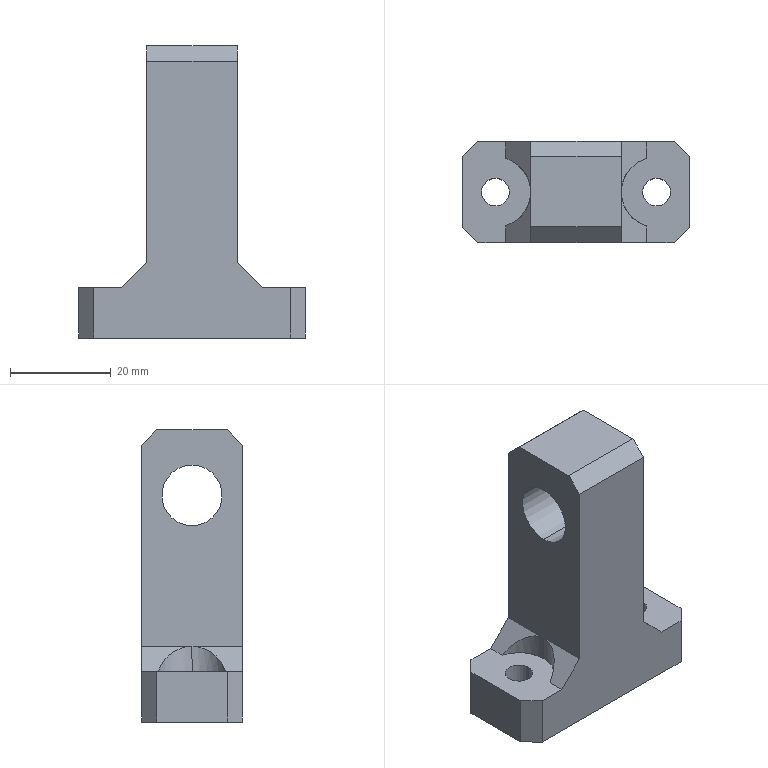Component | SolidWorks | FlipMechanismA-08-1 | 1 solid | 29 faces | box 45 x 20 x 58 mm | volume 23722 mm3 | plane 20 | cylinder 9 | commonest cylinder face diameters 5.5 x4 14 x3 12 x2
build123d program:
from build123d import *

# Parameters (mm, degrees)
SKETCH1_W                         = 10
SKETCH1_H                         = 45
EXTRUDE1_DEPTH                    = 10
SKETCH4_W                         = 18
SKETCH4_H                         = 20
EXTRUDE3_DEPTH                    = 48
M12X1_25_TAPPED_HOLE1_D           = 10.8
CHAMFER1_SIZE                     = 3
CHAMFER2_SIZE                     = 5
CHAMFER3_SIZE                     = 3
M5_CLEARANCE_HOLE_1_D             = 5.5
M5_CLEARANCE_HOLE_1_DEPTH         = 15
M5_CLEARANCE_HOLE_1_TIP           = 1.652
SKETCH4_2_R                       = 7
CUT_EXTRUDE1_DEPTH                = 18
TAPPEDHOLEMAJORDIA_M12_DEPTH      = 59.44
TAPPEDHOLEMAJORDIA_M12_DEPTH_BACK = 59.44
SKETCH7_R                         = 6


with BuildPart() as part:
    # Sketch1 → Extrude1 (new, symmetric)
    with BuildSketch(Plane(origin=(0, 0, 0), x_dir=(1, 0, 0), z_dir=(0, 1, 0))):
        Rectangle(SKETCH1_W, SKETCH1_H)
    extrude(amount=EXTRUDE1_DEPTH, both=True)

    # Sketch4 → Extrude3 (add)
    with BuildSketch(Plane(origin=(5, 0, 0), x_dir=(0, 0, -1), z_dir=(1, 0, 0))):
        Rectangle(SKETCH4_W, SKETCH4_H)
    extrude(amount=EXTRUDE3_DEPTH)

    # M12x1.25 Tapped Hole1 (through all)
    with Locations(Plane.XY.offset(9)):
        with Locations((40, 0)):
            Hole(M12X1_25_TAPPED_HOLE1_D / 2)

    # Chamfer1
    chamfer1_edges = [part.edges().sort_by_distance(p)[0] for p in [
        (0, -10, 22.5),
        (0, 10, 22.5),
        (0, -10, -22.5),
        (0, 10, -22.5),
    ]]
    chamfer(chamfer1_edges, length=CHAMFER1_SIZE)

    # Chamfer2
    chamfer2_edges = [part.edges().sort_by_distance(p)[0] for p in [
        (5, 0, -9),
        (5, 0, 9),
    ]]
    chamfer(chamfer2_edges, length=CHAMFER2_SIZE)

    # Chamfer3
    chamfer3_edges = [part.edges().sort_by_distance(p)[0] for p in [
        (53, -10, 0),
        (53, 10, 0),
    ]]
    chamfer(chamfer3_edges, length=CHAMFER3_SIZE)

    # M5 Clearance Hole 1
    with Locations(Plane(origin=(-5, 0, -16), x_dir=(0, 0, -1), z_dir=(-1, 0, 0))):
        with Locations((0, 0), (-32, 0)):
            Hole(M5_CLEARANCE_HOLE_1_D / 2, depth=M5_CLEARANCE_HOLE_1_DEPTH)
            with Locations((0, 0, -(M5_CLEARANCE_HOLE_1_DEPTH + M5_CLEARANCE_HOLE_1_TIP / 2))):  # 118° drill point
                Cone(0, M5_CLEARANCE_HOLE_1_D / 2, M5_CLEARANCE_HOLE_1_TIP, mode=Mode.SUBTRACT)

    # Sketch4_2 → Cut-Extrude1 (cut)
    with BuildSketch(Plane(origin=(5, 0, 0), x_dir=(0, 0, -1), z_dir=(1, 0, 0))):
        with Locations((16, 0)):
            Circle(SKETCH4_2_R)
        with Locations((-16, 0)):
            Circle(SKETCH4_2_R)
    extrude(amount=CUT_EXTRUDE1_DEPTH, mode=Mode.SUBTRACT)

    # Sketch7 → TappedHoleMajorDia_M12 (cut, two sides: drawn at the far end of the back side and taken through both)
    with BuildSketch(Plane.XY.offset(-TAPPEDHOLEMAJORDIA_M12_DEPTH_BACK)):
        with Locations((40, 0)):
            Circle(SKETCH7_R)
    extrude(amount=TAPPEDHOLEMAJORDIA_M12_DEPTH + TAPPEDHOLEMAJORDIA_M12_DEPTH_BACK, mode=Mode.SUBTRACT)


solid = part.part

# Placed as in the assembly
solid = solid.moved(Location((-99, 0, -40), (0, -90, 0)))
STEP:
#1=CARTESIAN_POINT('',(-4.252,-0.,-0.2362));
#2=VERTEX_POINT('',#1);
#3=CARTESIAN_POINT('',(-4.252,-0.,0.2362));
#4=VERTEX_POINT('',#3);
#5=CARTESIAN_POINT('',(-4.252,-0.,0.));
#6=DIRECTION('',(1.,0.,0.));
#7=DIRECTION('',(0.,1.,-0.));
#8=AXIS2_PLACEMENT_3D('',#5,#6,#7);
#9=CIRCLE('',#8,0.2362);
#10=EDGE_CURVE('',#2,#4,#9,.T.);
#11=ORIENTED_EDGE('',*,*,#10,.F.);
#12=CARTESIAN_POINT('',(-3.543,-0.,-0.2362));
#13=VERTEX_POINT('',#12);
#14=CARTESIAN_POINT('',(-4.783,-0.,-0.2362));
#15=DIRECTION('',(1.,-0.,0.));
#16=VECTOR('',#15,39.37);
#17=LINE('',#14,#16);
#18=EDGE_CURVE('',#2,#13,#17,.T.);
#19=ORIENTED_EDGE('',*,*,#18,.T.);
#20=CARTESIAN_POINT('',(-3.543,-0.,0.2362));
#21=VERTEX_POINT('',#20);
#22=CARTESIAN_POINT('',(-3.543,-0.,0.));
#23=DIRECTION('',(-1.,0.,-0.));
#24=DIRECTION('',(0.,-1.,0.));
#25=AXIS2_PLACEMENT_3D('',#22,#23,#24);
#26=CIRCLE('',#25,0.2362);
#27=EDGE_CURVE('',#21,#13,#26,.T.);
#28=ORIENTED_EDGE('',*,*,#27,.F.);
#29=CARTESIAN_POINT('',(-4.783,-0.,0.2362));
#30=DIRECTION('',(1.,-0.,0.));
#31=VECTOR('',#30,39.37);
#32=LINE('',#29,#31);
#33=EDGE_CURVE('',#4,#21,#32,.T.);
#34=ORIENTED_EDGE('',*,*,#33,.F.);
#35=EDGE_LOOP('',(#11,#19,#28,#34));
#36=FACE_OUTER_BOUND('',#35,.T.);
#37=CARTESIAN_POINT('',(-4.783,-0.,0.));
#38=DIRECTION('',(1.,-0.,0.));
#39=DIRECTION('',(0.,0.,1.));
#40=AXIS2_PLACEMENT_3D('',#37,#38,#39);
#41=CYLINDRICAL_SURFACE('',#40,0.2362);
#42=ADVANCED_FACE('',(#36),#41,.F.);
#43=CARTESIAN_POINT('',(-4.449,-0.2641,-1.378));
#44=VERTEX_POINT('',#43);
#45=CARTESIAN_POINT('',(-4.252,-0.,-1.181));
#46=VERTEX_POINT('',#45);
#47=CARTESIAN_POINT('',(-4.449,-0.2641,-1.378));
#48=CARTESIAN_POINT('',(-4.328,-0.228,-1.257));
#49=CARTESIAN_POINT('',(-4.252,-0.1265,-1.181));
#50=CARTESIAN_POINT('',(-4.252,-0.,-1.181));
#51=(BOUNDED_CURVE()B_SPLINE_CURVE(3,(#47,#48,#49,#50),.UNSPECIFIED.,.F.,.F.)B_SPLINE_CURVE_WITH_KNOTS((4,4),(1.861,3.142),.UNSPECIFIED.)CURVE()GEOMETRIC_REPRESENTATION_ITEM()RATIONAL_B_SPLINE_CURVE((1.,0.8679,0.8679,1.))REPRESENTATION_ITEM(''));
#52=EDGE_CURVE('',#44,#46,#51,.T.);
#53=ORIENTED_EDGE('',*,*,#52,.T.);
#54=CARTESIAN_POINT('',(-4.252,-0.,-1.378));
#55=VERTEX_POINT('',#54);
#56=CARTESIAN_POINT('',(-4.252,-0.,-0.6693));
#57=DIRECTION('',(0.,-0.,-1.));
#58=VECTOR('',#57,39.37);
#59=LINE('',#56,#58);
#60=EDGE_CURVE('',#46,#55,#59,.T.);
#61=ORIENTED_EDGE('',*,*,#60,.T.);
#62=CARTESIAN_POINT('',(-4.528,-0.,-1.378));
#63=DIRECTION('',(-0.,0.,1.));
#64=DIRECTION('',(-1.,0.,0.));
#65=AXIS2_PLACEMENT_3D('',#62,#63,#64);
#66=CIRCLE('',#65,0.2756);
#67=EDGE_CURVE('',#44,#55,#66,.T.);
#68=ORIENTED_EDGE('',*,*,#67,.F.);
#69=EDGE_LOOP('',(#53,#61,#68));
#70=FACE_OUTER_BOUND('',#69,.T.);
#71=CARTESIAN_POINT('',(-4.528,-0.,-0.6693));
#72=DIRECTION('',(0.,-0.,-1.));
#73=DIRECTION('',(1.,-0.,0.));
#74=AXIS2_PLACEMENT_3D('',#71,#72,#73);
#75=CYLINDRICAL_SURFACE('',#74,0.2756);
#76=ADVANCED_FACE('',(#70),#75,.F.);
#77=CARTESIAN_POINT('',(-4.636,-0.,-1.378));
#78=VERTEX_POINT('',#77);
#79=CARTESIAN_POINT('',(-4.419,-0.,-1.378));
#80=VERTEX_POINT('',#79);
#81=CARTESIAN_POINT('',(-4.528,-0.,-1.378));
#82=DIRECTION('',(0.,-0.,-1.));
#83=DIRECTION('',(1.,-0.,0.));
#84=AXIS2_PLACEMENT_3D('',#81,#82,#83);
#85=CIRCLE('',#84,0.1083);
#86=EDGE_CURVE('',#78,#80,#85,.T.);
#87=ORIENTED_EDGE('',*,*,#86,.F.);
#88=CARTESIAN_POINT('',(-4.636,-0.,-1.772));
#89=VERTEX_POINT('',#88);
#90=CARTESIAN_POINT('',(-4.636,-0.,-1.772));
#91=DIRECTION('',(0.,-0.,-1.));
#92=VECTOR('',#91,39.37);
#93=LINE('',#90,#92);
#94=EDGE_CURVE('',#78,#89,#93,.T.);
#95=ORIENTED_EDGE('',*,*,#94,.T.);
#96=CARTESIAN_POINT('',(-4.419,-0.,-1.772));
#97=VERTEX_POINT('',#96);
#98=CARTESIAN_POINT('',(-4.528,-0.,-1.772));
#99=DIRECTION('',(0.,-0.,-1.));
#100=DIRECTION('',(1.,-0.,0.));
#101=AXIS2_PLACEMENT_3D('',#98,#99,#100);
#102=CIRCLE('',#101,0.1083);
#103=EDGE_CURVE('',#89,#97,#102,.T.);
#104=ORIENTED_EDGE('',*,*,#103,.T.);
#105=CARTESIAN_POINT('',(-4.419,-0.,-1.772));
#106=DIRECTION('',(0.,-0.,-1.));
#107=VECTOR('',#106,39.37);
#108=LINE('',#105,#107);
#109=EDGE_CURVE('',#80,#97,#108,.T.);
#110=ORIENTED_EDGE('',*,*,#109,.F.);
#111=EDGE_LOOP('',(#87,#95,#104,#110));
#112=FACE_OUTER_BOUND('',#111,.T.);
#113=CARTESIAN_POINT('',(-4.528,-0.,-1.772));
#114=DIRECTION('',(0.,-0.,-1.));
#115=DIRECTION('',(1.,-0.,0.));
#116=AXIS2_PLACEMENT_3D('',#113,#114,#115);
#117=CYLINDRICAL_SURFACE('',#116,0.1083);
#118=ADVANCED_FACE('',(#112),#117,.F.);
#119=CARTESIAN_POINT('',(-3.376,-0.,-1.378));
#120=VERTEX_POINT('',#119);
#121=CARTESIAN_POINT('',(-3.159,-0.,-1.378));
#122=VERTEX_POINT('',#121);
#123=CARTESIAN_POINT('',(-3.268,-0.,-1.378));
#124=DIRECTION('',(0.,-0.,-1.));
#125=DIRECTION('',(1.,-0.,0.));
#126=AXIS2_PLACEMENT_3D('',#123,#124,#125);
#127=CIRCLE('',#126,0.1083);
#128=EDGE_CURVE('',#120,#122,#127,.T.);
#129=ORIENTED_EDGE('',*,*,#128,.F.);
#130=CARTESIAN_POINT('',(-3.376,-0.,-1.772));
#131=VERTEX_POINT('',#130);
#132=CARTESIAN_POINT('',(-3.376,-0.,-1.772));
#133=DIRECTION('',(0.,-0.,-1.));
#134=VECTOR('',#133,39.37);
#135=LINE('',#132,#134);
#136=EDGE_CURVE('',#120,#131,#135,.T.);
#137=ORIENTED_EDGE('',*,*,#136,.T.);
#138=CARTESIAN_POINT('',(-3.159,-0.,-1.772));
#139=VERTEX_POINT('',#138);
#140=CARTESIAN_POINT('',(-3.268,-0.,-1.772));
#141=DIRECTION('',(0.,-0.,-1.));
#142=DIRECTION('',(1.,-0.,0.));
#143=AXIS2_PLACEMENT_3D('',#140,#141,#142);
#144=CIRCLE('',#143,0.1083);
#145=EDGE_CURVE('',#131,#139,#144,.T.);
#146=ORIENTED_EDGE('',*,*,#145,.T.);
#147=CARTESIAN_POINT('',(-3.159,-0.,-1.772));
#148=DIRECTION('',(0.,-0.,-1.));
#149=VECTOR('',#148,39.37);
#150=LINE('',#147,#149);
#151=EDGE_CURVE('',#122,#139,#150,.T.);
#152=ORIENTED_EDGE('',*,*,#151,.F.);
#153=EDGE_LOOP('',(#129,#137,#146,#152));
#154=FACE_OUTER_BOUND('',#153,.T.);
#155=CARTESIAN_POINT('',(-3.268,-0.,-1.772));
#156=DIRECTION('',(0.,-0.,-1.));
#157=DIRECTION('',(1.,-0.,0.));
#158=AXIS2_PLACEMENT_3D('',#155,#156,#157);
#159=CYLINDRICAL_SURFACE('',#158,0.1083);
#160=ADVANCED_FACE('',(#154),#159,.F.);
#161=CARTESIAN_POINT('',(-3.346,0.2641,-1.378));
#162=VERTEX_POINT('',#161);
#163=CARTESIAN_POINT('',(-3.543,-0.,-1.181));
#164=VERTEX_POINT('',#163);
#165=CARTESIAN_POINT('',(-3.346,0.2641,-1.378));
#166=CARTESIAN_POINT('',(-3.468,0.228,-1.257));
#167=CARTESIAN_POINT('',(-3.543,0.1265,-1.181));
#168=CARTESIAN_POINT('',(-3.543,-0.,-1.181));
#169=(BOUNDED_CURVE()B_SPLINE_CURVE(3,(#165,#166,#167,#168),.UNSPECIFIED.,.F.,.T.)B_SPLINE_CURVE_WITH_KNOTS((4,4),(1.861,3.142),.UNSPECIFIED.)CURVE()GEOMETRIC_REPRESENTATION_ITEM()RATIONAL_B_SPLINE_CURVE((1.,0.8679,0.8679,1.))REPRESENTATION_ITEM(''));
#170=EDGE_CURVE('',#162,#164,#169,.T.);
#171=ORIENTED_EDGE('',*,*,#170,.F.);
#172=CARTESIAN_POINT('',(-3.346,0.3937,-1.378));
#173=VERTEX_POINT('',#172);
#174=CARTESIAN_POINT('',(-3.346,-0.3937,-1.378));
#175=DIRECTION('',(-0.,-1.,0.));
#176=VECTOR('',#175,39.37);
#177=LINE('',#174,#176);
#178=EDGE_CURVE('',#173,#162,#177,.T.);
#179=ORIENTED_EDGE('',*,*,#178,.F.);
#180=CARTESIAN_POINT('',(-3.543,0.3937,-1.181));
#181=VERTEX_POINT('',#180);
#182=CARTESIAN_POINT('',(-3.524,0.3937,-1.201));
#183=DIRECTION('',(0.7071,-0.,-0.7071));
#184=VECTOR('',#183,39.37);
#185=LINE('',#182,#184);
#186=EDGE_CURVE('',#181,#173,#185,.T.);
#187=ORIENTED_EDGE('',*,*,#186,.F.);
#188=CARTESIAN_POINT('',(-3.543,0.3937,-1.181));
#189=DIRECTION('',(0.,1.,-0.));
#190=VECTOR('',#189,39.37);
#191=LINE('',#188,#190);
#192=EDGE_CURVE('',#164,#181,#191,.T.);
#193=ORIENTED_EDGE('',*,*,#192,.F.);
#194=EDGE_LOOP('',(#171,#179,#187,#193));
#195=FACE_OUTER_BOUND('',#194,.T.);
#196=CARTESIAN_POINT('',(-3.543,-0.3937,-1.181));
#197=DIRECTION('',(0.7071,0.,0.7071));
#198=DIRECTION('',(-0.,-1.,0.));
#199=AXIS2_PLACEMENT_3D('',#196,#197,#198);
#200=PLANE('',#199);
#201=ADVANCED_FACE('',(#195),#200,.T.);
#202=CARTESIAN_POINT('',(-3.346,-0.2641,-1.378));
#203=VERTEX_POINT('',#202);
#204=CARTESIAN_POINT('',(-3.543,-0.,-1.181));
#205=CARTESIAN_POINT('',(-3.543,-0.1265,-1.181));
#206=CARTESIAN_POINT('',(-3.468,-0.228,-1.257));
#207=CARTESIAN_POINT('',(-3.346,-0.2641,-1.378));
#208=(BOUNDED_CURVE()B_SPLINE_CURVE(3,(#204,#205,#206,#207),.UNSPECIFIED.,.F.,.F.)B_SPLINE_CURVE_WITH_KNOTS((4,4),(3.142,4.423),.UNSPECIFIED.)CURVE()GEOMETRIC_REPRESENTATION_ITEM()RATIONAL_B_SPLINE_CURVE((1.,0.8679,0.8679,1.))REPRESENTATION_ITEM(''));
#209=EDGE_CURVE('',#164,#203,#208,.T.);
#210=ORIENTED_EDGE('',*,*,#209,.F.);
#211=CARTESIAN_POINT('',(-3.543,-0.3937,-1.181));
#212=VERTEX_POINT('',#211);
#213=CARTESIAN_POINT('',(-3.543,0.3937,-1.181));
#214=DIRECTION('',(0.,1.,-0.));
#215=VECTOR('',#214,39.37);
#216=LINE('',#213,#215);
#217=EDGE_CURVE('',#212,#164,#216,.T.);
#218=ORIENTED_EDGE('',*,*,#217,.F.);
#219=CARTESIAN_POINT('',(-3.346,-0.3937,-1.378));
#220=VERTEX_POINT('',#219);
#221=CARTESIAN_POINT('',(-3.543,-0.3937,-1.181));
#222=DIRECTION('',(-0.7071,0.,0.7071));
#223=VECTOR('',#222,39.37);
#224=LINE('',#221,#223);
#225=EDGE_CURVE('',#220,#212,#224,.T.);
#226=ORIENTED_EDGE('',*,*,#225,.F.);
#227=CARTESIAN_POINT('',(-3.346,-0.3937,-1.378));
#228=DIRECTION('',(-0.,-1.,0.));
#229=VECTOR('',#228,39.37);
#230=LINE('',#227,#229);
#231=EDGE_CURVE('',#203,#220,#230,.T.);
#232=ORIENTED_EDGE('',*,*,#231,.F.);
#233=EDGE_LOOP('',(#210,#218,#226,#232));
#234=FACE_OUTER_BOUND('',#233,.T.);
#235=CARTESIAN_POINT('',(-3.543,-0.3937,-1.181));
#236=DIRECTION('',(0.7071,0.,0.7071));
#237=DIRECTION('',(-0.,-1.,0.));
#238=AXIS2_PLACEMENT_3D('',#235,#236,#237);
#239=PLANE('',#238);
#240=ADVANCED_FACE('',(#234),#239,.T.);
#241=ORIENTED_EDGE('',*,*,#136,.F.);
#242=CARTESIAN_POINT('',(-3.268,-0.,-1.378));
#243=DIRECTION('',(0.,-0.,-1.));
#244=DIRECTION('',(1.,-0.,0.));
#245=AXIS2_PLACEMENT_3D('',#242,#243,#244);
#246=CIRCLE('',#245,0.1083);
#247=EDGE_CURVE('',#122,#120,#246,.T.);
#248=ORIENTED_EDGE('',*,*,#247,.F.);
#249=ORIENTED_EDGE('',*,*,#151,.T.);
#250=CARTESIAN_POINT('',(-3.268,-0.,-1.772));
#251=DIRECTION('',(0.,-0.,-1.));
#252=DIRECTION('',(1.,-0.,0.));
#253=AXIS2_PLACEMENT_3D('',#250,#251,#252);
#254=CIRCLE('',#253,0.1083);
#255=EDGE_CURVE('',#139,#131,#254,.T.);
#256=ORIENTED_EDGE('',*,*,#255,.T.);
#257=EDGE_LOOP('',(#241,#248,#249,#256));
#258=FACE_OUTER_BOUND('',#257,.T.);
#259=CARTESIAN_POINT('',(-3.268,-0.,-1.772));
#260=DIRECTION('',(0.,-0.,-1.));
#261=DIRECTION('',(1.,-0.,0.));
#262=AXIS2_PLACEMENT_3D('',#259,#260,#261);
#263=CYLINDRICAL_SURFACE('',#262,0.1083);
#264=ADVANCED_FACE('',(#258),#263,.F.);
#265=ORIENTED_EDGE('',*,*,#52,.F.);
#266=CARTESIAN_POINT('',(-4.449,-0.3937,-1.378));
#267=VERTEX_POINT('',#266);
#268=CARTESIAN_POINT('',(-4.449,0.3937,-1.378));
#269=DIRECTION('',(-0.,1.,-0.));
#270=VECTOR('',#269,39.37);
#271=LINE('',#268,#270);
#272=EDGE_CURVE('',#267,#44,#271,.T.);
#273=ORIENTED_EDGE('',*,*,#272,.F.);
#274=CARTESIAN_POINT('',(-4.252,-0.3937,-1.181));
#275=VERTEX_POINT('',#274);
#276=CARTESIAN_POINT('',(-4.252,-0.3937,-1.181));
#277=DIRECTION('',(-0.7071,-0.,-0.7071));
#278=VECTOR('',#277,39.37);
#279=LINE('',#276,#278);
#280=EDGE_CURVE('',#275,#267,#279,.T.);
#281=ORIENTED_EDGE('',*,*,#280,.F.);
#282=CARTESIAN_POINT('',(-4.252,-0.3937,-1.181));
#283=DIRECTION('',(0.,-1.,0.));
#284=VECTOR('',#283,39.37);
#285=LINE('',#282,#284);
#286=EDGE_CURVE('',#46,#275,#285,.T.);
#287=ORIENTED_EDGE('',*,*,#286,.F.);
#288=EDGE_LOOP('',(#265,#273,#281,#287));
#289=FACE_OUTER_BOUND('',#288,.T.);
#290=CARTESIAN_POINT('',(-4.252,-0.3937,-1.181));
#291=DIRECTION('',(-0.7071,0.,0.7071));
#292=DIRECTION('',(-0.,1.,-0.));
#293=AXIS2_PLACEMENT_3D('',#290,#291,#292);
#294=PLANE('',#293);
#295=ADVANCED_FACE('',(#289),#294,.T.);
#296=CARTESIAN_POINT('',(-4.449,0.2641,-1.378));
#297=VERTEX_POINT('',#296);
#298=CARTESIAN_POINT('',(-4.252,-0.,-1.181));
#299=CARTESIAN_POINT('',(-4.252,0.1265,-1.181));
#300=CARTESIAN_POINT('',(-4.328,0.228,-1.257));
#301=CARTESIAN_POINT('',(-4.449,0.2641,-1.378));
#302=(BOUNDED_CURVE()B_SPLINE_CURVE(3,(#298,#299,#300,#301),.UNSPECIFIED.,.F.,.F.)B_SPLINE_CURVE_WITH_KNOTS((4,4),(3.142,4.423),.UNSPECIFIED.)CURVE()GEOMETRIC_REPRESENTATION_ITEM()RATIONAL_B_SPLINE_CURVE((1.,0.8679,0.8679,1.))REPRESENTATION_ITEM(''));
#303=EDGE_CURVE('',#46,#297,#302,.T.);
#304=ORIENTED_EDGE('',*,*,#303,.F.);
#305=CARTESIAN_POINT('',(-4.252,0.3937,-1.181));
#306=VERTEX_POINT('',#305);
#307=CARTESIAN_POINT('',(-4.252,-0.3937,-1.181));
#308=DIRECTION('',(0.,-1.,0.));
#309=VECTOR('',#308,39.37);
#310=LINE('',#307,#309);
#311=EDGE_CURVE('',#306,#46,#310,.T.);
#312=ORIENTED_EDGE('',*,*,#311,.F.);
#313=CARTESIAN_POINT('',(-4.449,0.3937,-1.378));
#314=VERTEX_POINT('',#313);
#315=CARTESIAN_POINT('',(-4.272,0.3937,-1.201));
#316=DIRECTION('',(0.7071,0.,0.7071));
#317=VECTOR('',#316,39.37);
#318=LINE('',#315,#317);
#319=EDGE_CURVE('',#314,#306,#318,.T.);
#320=ORIENTED_EDGE('',*,*,#319,.F.);
#321=CARTESIAN_POINT('',(-4.449,0.3937,-1.378));
#322=DIRECTION('',(-0.,1.,-0.));
#323=VECTOR('',#322,39.37);
#324=LINE('',#321,#323);
#325=EDGE_CURVE('',#297,#314,#324,.T.);
#326=ORIENTED_EDGE('',*,*,#325,.F.);
#327=EDGE_LOOP('',(#304,#312,#320,#326));
#328=FACE_OUTER_BOUND('',#327,.T.);
#329=CARTESIAN_POINT('',(-4.252,-0.3937,-1.181));
#330=DIRECTION('',(-0.7071,0.,0.7071));
#331=DIRECTION('',(-0.,1.,-0.));
#332=AXIS2_PLACEMENT_3D('',#329,#330,#331);
#333=PLANE('',#332);
#334=ADVANCED_FACE('',(#328),#333,.T.);
#335=ORIENTED_EDGE('',*,*,#94,.F.);
#336=CARTESIAN_POINT('',(-4.528,-0.,-1.378));
#337=DIRECTION('',(0.,-0.,-1.));
#338=DIRECTION('',(1.,-0.,0.));
#339=AXIS2_PLACEMENT_3D('',#336,#337,#338);
#340=CIRCLE('',#339,0.1083);
#341=EDGE_CURVE('',#80,#78,#340,.T.);
#342=ORIENTED_EDGE('',*,*,#341,.F.);
#343=ORIENTED_EDGE('',*,*,#109,.T.);
#344=CARTESIAN_POINT('',(-4.528,-0.,-1.772));
#345=DIRECTION('',(0.,-0.,-1.));
#346=DIRECTION('',(1.,-0.,0.));
#347=AXIS2_PLACEMENT_3D('',#344,#345,#346);
#348=CIRCLE('',#347,0.1083);
#349=EDGE_CURVE('',#97,#89,#348,.T.);
#350=ORIENTED_EDGE('',*,*,#349,.T.);
#351=EDGE_LOOP('',(#335,#342,#343,#350));
#352=FACE_OUTER_BOUND('',#351,.T.);
#353=CARTESIAN_POINT('',(-4.528,-0.,-1.772));
#354=DIRECTION('',(0.,-0.,-1.));
#355=DIRECTION('',(1.,-0.,0.));
#356=AXIS2_PLACEMENT_3D('',#353,#354,#355);
#357=CYLINDRICAL_SURFACE('',#356,0.1083);
#358=ADVANCED_FACE('',(#352),#357,.F.);
#359=CARTESIAN_POINT('',(-3.268,-0.,-1.378));
#360=DIRECTION('',(-0.,0.,1.));
#361=DIRECTION('',(-1.,0.,0.));
#362=AXIS2_PLACEMENT_3D('',#359,#360,#361);
#363=CIRCLE('',#362,0.2756);
#364=EDGE_CURVE('',#162,#203,#363,.T.);
#365=ORIENTED_EDGE('',*,*,#364,.T.);
#366=ORIENTED_EDGE('',*,*,#231,.T.);
#367=CARTESIAN_POINT('',(-3.13,-0.3937,-1.378));
#368=VERTEX_POINT('',#367);
#369=CARTESIAN_POINT('',(-4.783,-0.3937,-1.378));
#370=DIRECTION('',(-1.,0.,-0.));
#371=VECTOR('',#370,39.37);
#372=LINE('',#369,#371);
#373=EDGE_CURVE('',#368,#220,#372,.T.);
#374=ORIENTED_EDGE('',*,*,#373,.F.);
#375=CARTESIAN_POINT('',(-3.012,-0.2756,-1.378));
#376=VERTEX_POINT('',#375);
#377=CARTESIAN_POINT('',(-3.13,-0.3937,-1.378));
#378=DIRECTION('',(0.7071,0.7071,0.));
#379=VECTOR('',#378,39.37);
#380=LINE('',#377,#379);
#381=EDGE_CURVE('',#368,#376,#380,.T.);
#382=ORIENTED_EDGE('',*,*,#381,.T.);
#383=CARTESIAN_POINT('',(-3.012,0.2756,-1.378));
#384=VERTEX_POINT('',#383);
#385=CARTESIAN_POINT('',(-3.012,-0.3937,-1.378));
#386=DIRECTION('',(0.,1.,-0.));
#387=VECTOR('',#386,39.37);
#388=LINE('',#385,#387);
#389=EDGE_CURVE('',#376,#384,#388,.T.);
#390=ORIENTED_EDGE('',*,*,#389,.T.);
#391=CARTESIAN_POINT('',(-3.13,0.3937,-1.378));
#392=VERTEX_POINT('',#391);
#393=CARTESIAN_POINT('',(-3.012,0.2756,-1.378));
#394=DIRECTION('',(-0.7071,0.7071,-0.));
#395=VECTOR('',#394,39.37);
#396=LINE('',#393,#395);
#397=EDGE_CURVE('',#384,#392,#396,.T.);
#398=ORIENTED_EDGE('',*,*,#397,.T.);
#399=CARTESIAN_POINT('',(-4.783,0.3937,-1.378));
#400=DIRECTION('',(-1.,0.,-0.));
#401=VECTOR('',#400,39.37);
#402=LINE('',#399,#401);
#403=EDGE_CURVE('',#392,#173,#402,.T.);
#404=ORIENTED_EDGE('',*,*,#403,.T.);
#405=ORIENTED_EDGE('',*,*,#178,.T.);
#406=EDGE_LOOP('',(#365,#366,#374,#382,#390,#398,#404,#405));
#407=FACE_OUTER_BOUND('',#406,.T.);
#408=ORIENTED_EDGE('',*,*,#247,.T.);
#409=ORIENTED_EDGE('',*,*,#128,.T.);
#410=EDGE_LOOP('',(#408,#409));
#411=FACE_BOUND('',#410,.T.);
#412=CARTESIAN_POINT('',(-4.783,-0.3937,-1.378));
#413=DIRECTION('',(0.,-0.,-1.));
#414=DIRECTION('',(1.,-0.,0.));
#415=AXIS2_PLACEMENT_3D('',#412,#413,#414);
#416=PLANE('',#415);
#417=ADVANCED_FACE('',(#407,#411),#416,.F.);
#418=ORIENTED_EDGE('',*,*,#67,.T.);
#419=CARTESIAN_POINT('',(-4.528,-0.,-1.378));
#420=DIRECTION('',(-0.,0.,1.));
#421=DIRECTION('',(-1.,0.,0.));
#422=AXIS2_PLACEMENT_3D('',#419,#420,#421);
#423=CIRCLE('',#422,0.2756);
#424=EDGE_CURVE('',#55,#297,#423,.T.);
#425=ORIENTED_EDGE('',*,*,#424,.T.);
#426=ORIENTED_EDGE('',*,*,#325,.T.);
#427=CARTESIAN_POINT('',(-4.665,0.3937,-1.378));
#428=VERTEX_POINT('',#427);
#429=CARTESIAN_POINT('',(-4.783,0.3937,-1.378));
#430=DIRECTION('',(-1.,0.,-0.));
#431=VECTOR('',#430,39.37);
#432=LINE('',#429,#431);
#433=EDGE_CURVE('',#314,#428,#432,.T.);
#434=ORIENTED_EDGE('',*,*,#433,.T.);
#435=CARTESIAN_POINT('',(-4.783,0.2756,-1.378));
#436=VERTEX_POINT('',#435);
#437=CARTESIAN_POINT('',(-4.783,0.2756,-1.378));
#438=DIRECTION('',(-0.7071,-0.7071,-0.));
#439=VECTOR('',#438,39.37);
#440=LINE('',#437,#439);
#441=EDGE_CURVE('',#428,#436,#440,.T.);
#442=ORIENTED_EDGE('',*,*,#441,.T.);
#443=CARTESIAN_POINT('',(-4.783,-0.2756,-1.378));
#444=VERTEX_POINT('',#443);
#445=CARTESIAN_POINT('',(-4.783,-0.3937,-1.378));
#446=DIRECTION('',(0.,1.,-0.));
#447=VECTOR('',#446,39.37);
#448=LINE('',#445,#447);
#449=EDGE_CURVE('',#444,#436,#448,.T.);
#450=ORIENTED_EDGE('',*,*,#449,.F.);
#451=CARTESIAN_POINT('',(-4.665,-0.3937,-1.378));
#452=VERTEX_POINT('',#451);
#453=CARTESIAN_POINT('',(-4.665,-0.3937,-1.378));
#454=DIRECTION('',(0.7071,-0.7071,0.));
#455=VECTOR('',#454,39.37);
#456=LINE('',#453,#455);
#457=EDGE_CURVE('',#444,#452,#456,.T.);
#458=ORIENTED_EDGE('',*,*,#457,.T.);
#459=CARTESIAN_POINT('',(-4.783,-0.3937,-1.378));
#460=DIRECTION('',(-1.,0.,-0.));
#461=VECTOR('',#460,39.37);
#462=LINE('',#459,#461);
#463=EDGE_CURVE('',#267,#452,#462,.T.);
#464=ORIENTED_EDGE('',*,*,#463,.F.);
#465=ORIENTED_EDGE('',*,*,#272,.T.);
#466=EDGE_LOOP('',(#418,#425,#426,#434,#442,#450,#458,#464,#465));
#467=FACE_OUTER_BOUND('',#466,.T.);
#468=ORIENTED_EDGE('',*,*,#341,.T.);
#469=ORIENTED_EDGE('',*,*,#86,.T.);
#470=EDGE_LOOP('',(#468,#469));
#471=FACE_BOUND('',#470,.T.);
#472=CARTESIAN_POINT('',(-4.783,-0.3937,-1.378));
#473=DIRECTION('',(0.,-0.,-1.));
#474=DIRECTION('',(1.,-0.,0.));
#475=AXIS2_PLACEMENT_3D('',#472,#473,#474);
#476=PLANE('',#475);
#477=ADVANCED_FACE('',(#467,#471),#476,.F.);
#478=ORIENTED_EDGE('',*,*,#349,.F.);
#479=ORIENTED_EDGE('',*,*,#103,.F.);
#480=EDGE_LOOP('',(#478,#479));
#481=FACE_BOUND('',#480,.T.);
#482=ORIENTED_EDGE('',*,*,#255,.F.);
#483=ORIENTED_EDGE('',*,*,#145,.F.);
#484=EDGE_LOOP('',(#482,#483));
#485=FACE_BOUND('',#484,.T.);
#486=CARTESIAN_POINT('',(-4.665,0.3937,-1.772));
#487=VERTEX_POINT('',#486);
#488=CARTESIAN_POINT('',(-3.13,0.3937,-1.772));
#489=VERTEX_POINT('',#488);
#490=CARTESIAN_POINT('',(-4.783,0.3937,-1.772));
#491=DIRECTION('',(1.,-0.,0.));
#492=VECTOR('',#491,39.37);
#493=LINE('',#490,#492);
#494=EDGE_CURVE('',#487,#489,#493,.T.);
#495=ORIENTED_EDGE('',*,*,#494,.T.);
#496=CARTESIAN_POINT('',(-3.012,0.2756,-1.772));
#497=VERTEX_POINT('',#496);
#498=CARTESIAN_POINT('',(-3.012,0.2756,-1.772));
#499=DIRECTION('',(0.7071,-0.7071,0.));
#500=VECTOR('',#499,39.37);
#501=LINE('',#498,#500);
#502=EDGE_CURVE('',#489,#497,#501,.T.);
#503=ORIENTED_EDGE('',*,*,#502,.T.);
#504=CARTESIAN_POINT('',(-3.012,-0.2756,-1.772));
#505=VERTEX_POINT('',#504);
#506=CARTESIAN_POINT('',(-3.012,-0.3937,-1.772));
#507=DIRECTION('',(0.,1.,-0.));
#508=VECTOR('',#507,39.37);
#509=LINE('',#506,#508);
#510=EDGE_CURVE('',#505,#497,#509,.T.);
#511=ORIENTED_EDGE('',*,*,#510,.F.);
#512=CARTESIAN_POINT('',(-3.13,-0.3937,-1.772));
#513=VERTEX_POINT('',#512);
#514=CARTESIAN_POINT('',(-3.13,-0.3937,-1.772));
#515=DIRECTION('',(-0.7071,-0.7071,-0.));
#516=VECTOR('',#515,39.37);
#517=LINE('',#514,#516);
#518=EDGE_CURVE('',#505,#513,#517,.T.);
#519=ORIENTED_EDGE('',*,*,#518,.T.);
#520=CARTESIAN_POINT('',(-4.665,-0.3937,-1.772));
#521=VERTEX_POINT('',#520);
#522=CARTESIAN_POINT('',(-4.783,-0.3937,-1.772));
#523=DIRECTION('',(1.,-0.,0.));
#524=VECTOR('',#523,39.37);
#525=LINE('',#522,#524);
#526=EDGE_CURVE('',#521,#513,#525,.T.);
#527=ORIENTED_EDGE('',*,*,#526,.F.);
#528=CARTESIAN_POINT('',(-4.783,-0.2756,-1.772));
#529=VERTEX_POINT('',#528);
#530=CARTESIAN_POINT('',(-4.665,-0.3937,-1.772));
#531=DIRECTION('',(-0.7071,0.7071,-0.));
#532=VECTOR('',#531,39.37);
#533=LINE('',#530,#532);
#534=EDGE_CURVE('',#521,#529,#533,.T.);
#535=ORIENTED_EDGE('',*,*,#534,.T.);
#536=CARTESIAN_POINT('',(-4.783,0.2756,-1.772));
#537=VERTEX_POINT('',#536);
#538=CARTESIAN_POINT('',(-4.783,-0.3937,-1.772));
#539=DIRECTION('',(0.,1.,-0.));
#540=VECTOR('',#539,39.37);
#541=LINE('',#538,#540);
#542=EDGE_CURVE('',#529,#537,#541,.T.);
#543=ORIENTED_EDGE('',*,*,#542,.T.);
#544=CARTESIAN_POINT('',(-4.783,0.2756,-1.772));
#545=DIRECTION('',(0.7071,0.7071,0.));
#546=VECTOR('',#545,39.37);
#547=LINE('',#544,#546);
#548=EDGE_CURVE('',#537,#487,#547,.T.);
#549=ORIENTED_EDGE('',*,*,#548,.T.);
#550=EDGE_LOOP('',(#495,#503,#511,#519,#527,#535,#543,#549));
#551=FACE_OUTER_BOUND('',#550,.T.);
#552=CARTESIAN_POINT('',(-4.783,-0.3937,-1.772));
#553=DIRECTION('',(-0.,0.,1.));
#554=DIRECTION('',(-1.,0.,-0.));
#555=AXIS2_PLACEMENT_3D('',#552,#553,#554);
#556=PLANE('',#555);
#557=ADVANCED_FACE('',(#481,#485,#551),#556,.F.);
#558=ORIENTED_EDGE('',*,*,#510,.T.);
#559=CARTESIAN_POINT('',(-3.012,0.2756,-1.772));
#560=DIRECTION('',(-0.,0.,1.));
#561=VECTOR('',#560,39.37);
#562=LINE('',#559,#561);
#563=EDGE_CURVE('',#497,#384,#562,.T.);
#564=ORIENTED_EDGE('',*,*,#563,.T.);
#565=ORIENTED_EDGE('',*,*,#389,.F.);
#566=CARTESIAN_POINT('',(-3.012,-0.2756,-1.772));
#567=DIRECTION('',(0.,-0.,-1.));
#568=VECTOR('',#567,39.37);
#569=LINE('',#566,#568);
#570=EDGE_CURVE('',#376,#505,#569,.T.);
#571=ORIENTED_EDGE('',*,*,#570,.T.);
#572=EDGE_LOOP('',(#558,#564,#565,#571));
#573=FACE_OUTER_BOUND('',#572,.T.);
#574=CARTESIAN_POINT('',(-3.012,-0.3937,-1.772));
#575=DIRECTION('',(-1.,0.,-0.));
#576=DIRECTION('',(0.,-0.,-1.));
#577=AXIS2_PLACEMENT_3D('',#574,#575,#576);
#578=PLANE('',#577);
#579=ADVANCED_FACE('',(#573),#578,.F.);
#580=ORIENTED_EDGE('',*,*,#449,.T.);
#581=CARTESIAN_POINT('',(-4.783,0.2756,-1.772));
#582=DIRECTION('',(0.,-0.,-1.));
#583=VECTOR('',#582,39.37);
#584=LINE('',#581,#583);
#585=EDGE_CURVE('',#436,#537,#584,.T.);
#586=ORIENTED_EDGE('',*,*,#585,.T.);
#587=ORIENTED_EDGE('',*,*,#542,.F.);
#588=CARTESIAN_POINT('',(-4.783,-0.2756,-1.378));
#589=DIRECTION('',(-0.,0.,1.));
#590=VECTOR('',#589,39.37);
#591=LINE('',#588,#590);
#592=EDGE_CURVE('',#529,#444,#591,.T.);
#593=ORIENTED_EDGE('',*,*,#592,.T.);
#594=EDGE_LOOP('',(#580,#586,#587,#593));
#595=FACE_OUTER_BOUND('',#594,.T.);
#596=CARTESIAN_POINT('',(-4.783,-0.3937,-1.772));
#597=DIRECTION('',(1.,-0.,0.));
#598=DIRECTION('',(-0.,0.,1.));
#599=AXIS2_PLACEMENT_3D('',#596,#597,#598);
#600=PLANE('',#599);
#601=ADVANCED_FACE('',(#595),#600,.F.);
#602=CARTESIAN_POINT('',(-3.543,-0.3937,0.3937));
#603=VERTEX_POINT('',#602);
#604=CARTESIAN_POINT('',(-3.543,-0.3937,0.5118));
#605=DIRECTION('',(0.,-0.,-1.));
#606=VECTOR('',#605,39.37);
#607=LINE('',#604,#606);
#608=EDGE_CURVE('',#603,#212,#607,.T.);
#609=ORIENTED_EDGE('',*,*,#608,.F.);
#610=CARTESIAN_POINT('',(-4.252,-0.3937,0.3937));
#611=VERTEX_POINT('',#610);
#612=CARTESIAN_POINT('',(-3.898,-0.3937,0.3937));
#613=DIRECTION('',(-1.,0.,-0.));
#614=VECTOR('',#613,39.37);
#615=LINE('',#612,#614);
#616=EDGE_CURVE('',#603,#611,#615,.T.);
#617=ORIENTED_EDGE('',*,*,#616,.T.);
#618=CARTESIAN_POINT('',(-4.252,-0.3937,0.5118));
#619=DIRECTION('',(0.,-0.,-1.));
#620=VECTOR('',#619,39.37);
#621=LINE('',#618,#620);
#622=EDGE_CURVE('',#611,#275,#621,.T.);
#623=ORIENTED_EDGE('',*,*,#622,.T.);
#624=ORIENTED_EDGE('',*,*,#280,.T.);
#625=ORIENTED_EDGE('',*,*,#463,.T.);
#626=CARTESIAN_POINT('',(-4.665,-0.3937,-1.772));
#627=DIRECTION('',(0.,-0.,-1.));
#628=VECTOR('',#627,39.37);
#629=LINE('',#626,#628);
#630=EDGE_CURVE('',#452,#521,#629,.T.);
#631=ORIENTED_EDGE('',*,*,#630,.T.);
#632=ORIENTED_EDGE('',*,*,#526,.T.);
#633=CARTESIAN_POINT('',(-3.13,-0.3937,-1.378));
#634=DIRECTION('',(-0.,0.,1.));
#635=VECTOR('',#634,39.37);
#636=LINE('',#633,#635);
#637=EDGE_CURVE('',#513,#368,#636,.T.);
#638=ORIENTED_EDGE('',*,*,#637,.T.);
#639=ORIENTED_EDGE('',*,*,#373,.T.);
#640=ORIENTED_EDGE('',*,*,#225,.T.);
#641=EDGE_LOOP('',(#609,#617,#623,#624,#625,#631,#632,#638,#639,#640));
#642=FACE_OUTER_BOUND('',#641,.T.);
#643=CARTESIAN_POINT('',(-3.898,-0.3937,-1.575));
#644=DIRECTION('',(-0.,-1.,0.));
#645=DIRECTION('',(1.,-0.,0.));
#646=AXIS2_PLACEMENT_3D('',#643,#644,#645);
#647=PLANE('',#646);
#648=ADVANCED_FACE('',(#642),#647,.T.);
#649=CARTESIAN_POINT('',(-4.252,0.3937,0.3937));
#650=VERTEX_POINT('',#649);
#651=CARTESIAN_POINT('',(-4.252,0.3937,0.5118));
#652=DIRECTION('',(0.,-0.,-1.));
#653=VECTOR('',#652,39.37);
#654=LINE('',#651,#653);
#655=EDGE_CURVE('',#650,#306,#654,.T.);
#656=ORIENTED_EDGE('',*,*,#655,.F.);
#657=CARTESIAN_POINT('',(-3.543,0.3937,0.3937));
#658=VERTEX_POINT('',#657);
#659=CARTESIAN_POINT('',(-3.543,0.3937,0.3937));
#660=DIRECTION('',(1.,-0.,0.));
#661=VECTOR('',#660,39.37);
#662=LINE('',#659,#661);
#663=EDGE_CURVE('',#650,#658,#662,.T.);
#664=ORIENTED_EDGE('',*,*,#663,.T.);
#665=CARTESIAN_POINT('',(-3.543,0.3937,0.5118));
#666=DIRECTION('',(0.,-0.,-1.));
#667=VECTOR('',#666,39.37);
#668=LINE('',#665,#667);
#669=EDGE_CURVE('',#658,#181,#668,.T.);
#670=ORIENTED_EDGE('',*,*,#669,.T.);
#671=ORIENTED_EDGE('',*,*,#186,.T.);
#672=ORIENTED_EDGE('',*,*,#403,.F.);
#673=CARTESIAN_POINT('',(-3.13,0.3937,-1.575));
#674=DIRECTION('',(0.,-0.,-1.));
#675=VECTOR('',#674,39.37);
#676=LINE('',#673,#675);
#677=EDGE_CURVE('',#392,#489,#676,.T.);
#678=ORIENTED_EDGE('',*,*,#677,.T.);
#679=ORIENTED_EDGE('',*,*,#494,.F.);
#680=CARTESIAN_POINT('',(-4.665,0.3937,-1.575));
#681=DIRECTION('',(-0.,0.,1.));
#682=VECTOR('',#681,39.37);
#683=LINE('',#680,#682);
#684=EDGE_CURVE('',#487,#428,#683,.T.);
#685=ORIENTED_EDGE('',*,*,#684,.T.);
#686=ORIENTED_EDGE('',*,*,#433,.F.);
#687=ORIENTED_EDGE('',*,*,#319,.T.);
#688=EDGE_LOOP('',(#656,#664,#670,#671,#672,#678,#679,#685,#686,#687));
#689=FACE_OUTER_BOUND('',#688,.T.);
#690=CARTESIAN_POINT('',(-3.898,0.3937,-1.575));
#691=DIRECTION('',(-0.,-1.,0.));
#692=DIRECTION('',(1.,-0.,0.));
#693=AXIS2_PLACEMENT_3D('',#690,#691,#692);
#694=PLANE('',#693);
#695=ADVANCED_FACE('',(#689),#694,.F.);
#696=ORIENTED_EDGE('',*,*,#27,.T.);
#697=CARTESIAN_POINT('',(-3.543,-0.,0.));
#698=DIRECTION('',(-1.,0.,-0.));
#699=DIRECTION('',(0.,-1.,0.));
#700=AXIS2_PLACEMENT_3D('',#697,#698,#699);
#701=CIRCLE('',#700,0.2362);
#702=EDGE_CURVE('',#13,#21,#701,.T.);
#703=ORIENTED_EDGE('',*,*,#702,.T.);
#704=EDGE_LOOP('',(#696,#703));
#705=FACE_BOUND('',#704,.T.);
#706=ORIENTED_EDGE('',*,*,#669,.F.);
#707=CARTESIAN_POINT('',(-3.543,0.2756,0.5118));
#708=VERTEX_POINT('',#707);
#709=CARTESIAN_POINT('',(-3.543,0.2756,0.5118));
#710=DIRECTION('',(-0.,-0.7071,0.7071));
#711=VECTOR('',#710,39.37);
#712=LINE('',#709,#711);
#713=EDGE_CURVE('',#658,#708,#712,.T.);
#714=ORIENTED_EDGE('',*,*,#713,.T.);
#715=CARTESIAN_POINT('',(-3.543,-0.2756,0.5118));
#716=VERTEX_POINT('',#715);
#717=CARTESIAN_POINT('',(-3.543,-0.3937,0.5118));
#718=DIRECTION('',(0.,1.,-0.));
#719=VECTOR('',#718,39.37);
#720=LINE('',#717,#719);
#721=EDGE_CURVE('',#716,#708,#720,.T.);
#722=ORIENTED_EDGE('',*,*,#721,.F.);
#723=CARTESIAN_POINT('',(-3.543,-0.2756,0.5118));
#724=DIRECTION('',(0.,-0.7071,-0.7071));
#725=VECTOR('',#724,39.37);
#726=LINE('',#723,#725);
#727=EDGE_CURVE('',#716,#603,#726,.T.);
#728=ORIENTED_EDGE('',*,*,#727,.T.);
#729=ORIENTED_EDGE('',*,*,#608,.T.);
#730=ORIENTED_EDGE('',*,*,#217,.T.);
#731=ORIENTED_EDGE('',*,*,#192,.T.);
#732=EDGE_LOOP('',(#706,#714,#722,#728,#729,#730,#731));
#733=FACE_OUTER_BOUND('',#732,.T.);
#734=CARTESIAN_POINT('',(-3.543,-0.3937,0.5118));
#735=DIRECTION('',(-1.,0.,-0.));
#736=DIRECTION('',(-0.,-1.,0.));
#737=AXIS2_PLACEMENT_3D('',#734,#735,#736);
#738=PLANE('',#737);
#739=ADVANCED_FACE('',(#705,#733),#738,.F.);
#740=CARTESIAN_POINT('',(-4.252,-0.,0.));
#741=DIRECTION('',(1.,0.,0.));
#742=DIRECTION('',(0.,1.,-0.));
#743=AXIS2_PLACEMENT_3D('',#740,#741,#742);
#744=CIRCLE('',#743,0.2362);
#745=EDGE_CURVE('',#4,#2,#744,.T.);
#746=ORIENTED_EDGE('',*,*,#745,.T.);
#747=ORIENTED_EDGE('',*,*,#10,.T.);
#748=EDGE_LOOP('',(#746,#747));
#749=FACE_BOUND('',#748,.T.);
#750=CARTESIAN_POINT('',(-4.252,0.2756,0.5118));
#751=VERTEX_POINT('',#750);
#752=CARTESIAN_POINT('',(-4.252,-0.2756,0.5118));
#753=VERTEX_POINT('',#752);
#754=CARTESIAN_POINT('',(-4.252,-0.3937,0.5118));
#755=DIRECTION('',(0.,-1.,0.));
#756=VECTOR('',#755,39.37);
#757=LINE('',#754,#756);
#758=EDGE_CURVE('',#751,#753,#757,.T.);
#759=ORIENTED_EDGE('',*,*,#758,.F.);
#760=CARTESIAN_POINT('',(-4.252,0.2756,0.5118));
#761=DIRECTION('',(0.,0.7071,-0.7071));
#762=VECTOR('',#761,39.37);
#763=LINE('',#760,#762);
#764=EDGE_CURVE('',#751,#650,#763,.T.);
#765=ORIENTED_EDGE('',*,*,#764,.T.);
#766=ORIENTED_EDGE('',*,*,#655,.T.);
#767=ORIENTED_EDGE('',*,*,#311,.T.);
#768=ORIENTED_EDGE('',*,*,#286,.T.);
#769=ORIENTED_EDGE('',*,*,#622,.F.);
#770=CARTESIAN_POINT('',(-4.252,-0.2756,0.5118));
#771=DIRECTION('',(-0.,0.7071,0.7071));
#772=VECTOR('',#771,39.37);
#773=LINE('',#770,#772);
#774=EDGE_CURVE('',#611,#753,#773,.T.);
#775=ORIENTED_EDGE('',*,*,#774,.T.);
#776=EDGE_LOOP('',(#759,#765,#766,#767,#768,#769,#775));
#777=FACE_OUTER_BOUND('',#776,.T.);
#778=CARTESIAN_POINT('',(-4.252,-0.3937,0.5118));
#779=DIRECTION('',(1.,0.,0.));
#780=DIRECTION('',(-0.,1.,-0.));
#781=AXIS2_PLACEMENT_3D('',#778,#779,#780);
#782=PLANE('',#781);
#783=ADVANCED_FACE('',(#749,#777),#782,.F.);
#784=ORIENTED_EDGE('',*,*,#721,.T.);
#785=CARTESIAN_POINT('',(-4.252,0.2756,0.5118));
#786=DIRECTION('',(-1.,0.,-0.));
#787=VECTOR('',#786,39.37);
#788=LINE('',#785,#787);
#789=EDGE_CURVE('',#708,#751,#788,.T.);
#790=ORIENTED_EDGE('',*,*,#789,.T.);
#791=ORIENTED_EDGE('',*,*,#758,.T.);
#792=CARTESIAN_POINT('',(-3.898,-0.2756,0.5118));
#793=DIRECTION('',(1.,-0.,0.));
#794=VECTOR('',#793,39.37);
#795=LINE('',#792,#794);
#796=EDGE_CURVE('',#753,#716,#795,.T.);
#797=ORIENTED_EDGE('',*,*,#796,.T.);
#798=EDGE_LOOP('',(#784,#790,#791,#797));
#799=FACE_OUTER_BOUND('',#798,.T.);
#800=CARTESIAN_POINT('',(-3.898,-0.,0.5118));
#801=DIRECTION('',(-0.,0.,1.));
#802=DIRECTION('',(-1.,0.,-0.));
#803=AXIS2_PLACEMENT_3D('',#800,#801,#802);
#804=PLANE('',#803);
#805=ADVANCED_FACE('',(#799),#804,.T.);
#806=ORIENTED_EDGE('',*,*,#502,.F.);
#807=ORIENTED_EDGE('',*,*,#677,.F.);
#808=ORIENTED_EDGE('',*,*,#397,.F.);
#809=ORIENTED_EDGE('',*,*,#563,.F.);
#810=EDGE_LOOP('',(#806,#807,#808,#809));
#811=FACE_OUTER_BOUND('',#810,.T.);
#812=CARTESIAN_POINT('',(-3.012,0.2756,-1.772));
#813=DIRECTION('',(-0.7071,-0.7071,-0.));
#814=DIRECTION('',(-0.,0.,1.));
#815=AXIS2_PLACEMENT_3D('',#812,#813,#814);
#816=PLANE('',#815);
#817=ADVANCED_FACE('',(#811),#816,.F.);
#818=ORIENTED_EDGE('',*,*,#518,.F.);
#819=ORIENTED_EDGE('',*,*,#570,.F.);
#820=ORIENTED_EDGE('',*,*,#381,.F.);
#821=ORIENTED_EDGE('',*,*,#637,.F.);
#822=EDGE_LOOP('',(#818,#819,#820,#821));
#823=FACE_OUTER_BOUND('',#822,.T.);
#824=CARTESIAN_POINT('',(-3.13,-0.3937,-1.575));
#825=DIRECTION('',(0.7071,-0.7071,0.));
#826=DIRECTION('',(0.,-0.,-1.));
#827=AXIS2_PLACEMENT_3D('',#824,#825,#826);
#828=PLANE('',#827);
#829=ADVANCED_FACE('',(#823),#828,.T.);
#830=ORIENTED_EDGE('',*,*,#441,.F.);
#831=ORIENTED_EDGE('',*,*,#684,.F.);
#832=ORIENTED_EDGE('',*,*,#548,.F.);
#833=ORIENTED_EDGE('',*,*,#585,.F.);
#834=EDGE_LOOP('',(#830,#831,#832,#833));
#835=FACE_OUTER_BOUND('',#834,.T.);
#836=CARTESIAN_POINT('',(-4.783,0.2756,-1.772));
#837=DIRECTION('',(0.7071,-0.7071,0.));
#838=DIRECTION('',(0.,-0.,-1.));
#839=AXIS2_PLACEMENT_3D('',#836,#837,#838);
#840=PLANE('',#839);
#841=ADVANCED_FACE('',(#835),#840,.F.);
#842=ORIENTED_EDGE('',*,*,#457,.F.);
#843=ORIENTED_EDGE('',*,*,#592,.F.);
#844=ORIENTED_EDGE('',*,*,#534,.F.);
#845=ORIENTED_EDGE('',*,*,#630,.F.);
#846=EDGE_LOOP('',(#842,#843,#844,#845));
#847=FACE_OUTER_BOUND('',#846,.T.);
#848=CARTESIAN_POINT('',(-4.665,-0.3937,-1.575));
#849=DIRECTION('',(-0.7071,-0.7071,-0.));
#850=DIRECTION('',(-0.,0.,1.));
#851=AXIS2_PLACEMENT_3D('',#848,#849,#850);
#852=PLANE('',#851);
#853=ADVANCED_FACE('',(#847),#852,.T.);
#854=ORIENTED_EDGE('',*,*,#713,.F.);
#855=ORIENTED_EDGE('',*,*,#663,.F.);
#856=ORIENTED_EDGE('',*,*,#764,.F.);
#857=ORIENTED_EDGE('',*,*,#789,.F.);
#858=EDGE_LOOP('',(#854,#855,#856,#857));
#859=FACE_OUTER_BOUND('',#858,.T.);
#860=CARTESIAN_POINT('',(-3.898,0.2756,0.5118));
#861=DIRECTION('',(-0.,0.7071,0.7071));
#862=DIRECTION('',(1.,-0.,0.));
#863=AXIS2_PLACEMENT_3D('',#860,#861,#862);
#864=PLANE('',#863);
#865=ADVANCED_FACE('',(#859),#864,.T.);
#866=ORIENTED_EDGE('',*,*,#774,.F.);
#867=ORIENTED_EDGE('',*,*,#616,.F.);
#868=ORIENTED_EDGE('',*,*,#727,.F.);
#869=ORIENTED_EDGE('',*,*,#796,.F.);
#870=EDGE_LOOP('',(#866,#867,#868,#869));
#871=FACE_OUTER_BOUND('',#870,.T.);
#872=CARTESIAN_POINT('',(-3.898,-0.2756,0.5118));
#873=DIRECTION('',(0.,0.7071,-0.7071));
#874=DIRECTION('',(1.,-0.,0.));
#875=AXIS2_PLACEMENT_3D('',#872,#873,#874);
#876=PLANE('',#875);
#877=ADVANCED_FACE('',(#871),#876,.F.);
#878=ORIENTED_EDGE('',*,*,#60,.F.);
#879=ORIENTED_EDGE('',*,*,#303,.T.);
#880=ORIENTED_EDGE('',*,*,#424,.F.);
#881=EDGE_LOOP('',(#878,#879,#880));
#882=FACE_OUTER_BOUND('',#881,.T.);
#883=CARTESIAN_POINT('',(-4.528,-0.,-0.6693));
#884=DIRECTION('',(0.,-0.,-1.));
#885=DIRECTION('',(1.,-0.,0.));
#886=AXIS2_PLACEMENT_3D('',#883,#884,#885);
#887=CYLINDRICAL_SURFACE('',#886,0.2756);
#888=ADVANCED_FACE('',(#882),#887,.F.);
#889=ORIENTED_EDGE('',*,*,#170,.T.);
#890=ORIENTED_EDGE('',*,*,#209,.T.);
#891=ORIENTED_EDGE('',*,*,#364,.F.);
#892=EDGE_LOOP('',(#889,#890,#891));
#893=FACE_OUTER_BOUND('',#892,.T.);
#894=CARTESIAN_POINT('',(-3.268,-0.,-0.6693));
#895=DIRECTION('',(0.,-0.,-1.));
#896=DIRECTION('',(1.,-0.,0.));
#897=AXIS2_PLACEMENT_3D('',#894,#895,#896);
#898=CYLINDRICAL_SURFACE('',#897,0.2756);
#899=ADVANCED_FACE('',(#893),#898,.F.);
#900=ORIENTED_EDGE('',*,*,#18,.F.);
#901=ORIENTED_EDGE('',*,*,#745,.F.);
#902=ORIENTED_EDGE('',*,*,#33,.T.);
#903=ORIENTED_EDGE('',*,*,#702,.F.);
#904=EDGE_LOOP('',(#900,#901,#902,#903));
#905=FACE_OUTER_BOUND('',#904,.T.);
#906=CARTESIAN_POINT('',(-4.783,-0.,0.));
#907=DIRECTION('',(1.,-0.,0.));
#908=DIRECTION('',(0.,0.,1.));
#909=AXIS2_PLACEMENT_3D('',#906,#907,#908);
#910=CYLINDRICAL_SURFACE('',#909,0.2362);
#911=ADVANCED_FACE('',(#905),#910,.F.);
#912=CLOSED_SHELL('',(#42,#76,#118,#160,#201,#240,#264,#295,#334,#358,#417,#477,#557,#579,#601,#648,#695,#739,#783,#805,#817,#829,#841,#853,#865,#877,#888,#899,#911));
#913=MANIFOLD_SOLID_BREP('',#912);
#914=CARTESIAN_POINT('',(0.,0.,0.));
#915=DIRECTION('',(0.,0.,1.));
#916=DIRECTION('',(1.,0.,0.));
#917=AXIS2_PLACEMENT_3D('',#914,#915,#916);
#918=(LENGTH_UNIT()NAMED_UNIT(*)SI_UNIT($,.METRE.));
#919=LENGTH_MEASURE_WITH_UNIT(LENGTH_MEASURE(0.0254),#918);
#920=DIMENSIONAL_EXPONENTS(1.,0.,0.,0.,0.,0.,0.);
#921=(CONVERSION_BASED_UNIT('',#919)LENGTH_UNIT()NAMED_UNIT(#920));
#922=UNCERTAINTY_MEASURE_WITH_UNIT(LENGTH_MEASURE(0.00001),#921,'','');
#923=(NAMED_UNIT(*)PLANE_ANGLE_UNIT()SI_UNIT($,.RADIAN.));
#924=(NAMED_UNIT(*)SI_UNIT($,.STERADIAN.)SOLID_ANGLE_UNIT());
#925=(GEOMETRIC_REPRESENTATION_CONTEXT(3)GLOBAL_UNCERTAINTY_ASSIGNED_CONTEXT((#922))GLOBAL_UNIT_ASSIGNED_CONTEXT((#921,#923,#924))REPRESENTATION_CONTEXT('',''));
#926=ADVANCED_BREP_SHAPE_REPRESENTATION('',(#913,#917),#925);
#927=COLOUR_RGB('',0.7922,0.8196,0.9333);
#928=FILL_AREA_STYLE_COLOUR('',#927);
#929=FILL_AREA_STYLE('',(#928));
#930=SURFACE_STYLE_FILL_AREA(#929);
#931=SURFACE_SIDE_STYLE('',(#930));
#932=SURFACE_STYLE_USAGE(.BOTH.,#931);
#933=PRESENTATION_STYLE_ASSIGNMENT((#932));
#934=STYLED_ITEM('',(#933),#913);
#935=PRESENTATION_LAYER_ASSIGNMENT('','',(#934));
#936=(LENGTH_UNIT()NAMED_UNIT(*)SI_UNIT($,.METRE.));
#937=LENGTH_MEASURE_WITH_UNIT(LENGTH_MEASURE(0.0254),#936);
#938=DIMENSIONAL_EXPONENTS(1.,0.,0.,0.,0.,0.,0.);
#939=(CONVERSION_BASED_UNIT('',#937)LENGTH_UNIT()NAMED_UNIT(#938));
#940=UNCERTAINTY_MEASURE_WITH_UNIT(LENGTH_MEASURE(0.00001),#939,'','');
#941=(NAMED_UNIT(*)PLANE_ANGLE_UNIT()SI_UNIT($,.RADIAN.));
#942=(NAMED_UNIT(*)SI_UNIT($,.STERADIAN.)SOLID_ANGLE_UNIT());
#943=(GEOMETRIC_REPRESENTATION_CONTEXT(3)GLOBAL_UNCERTAINTY_ASSIGNED_CONTEXT((#940))GLOBAL_UNIT_ASSIGNED_CONTEXT((#939,#941,#942))REPRESENTATION_CONTEXT('',''));
#944=MECHANICAL_DESIGN_GEOMETRIC_PRESENTATION_REPRESENTATION('',(#934),#943);